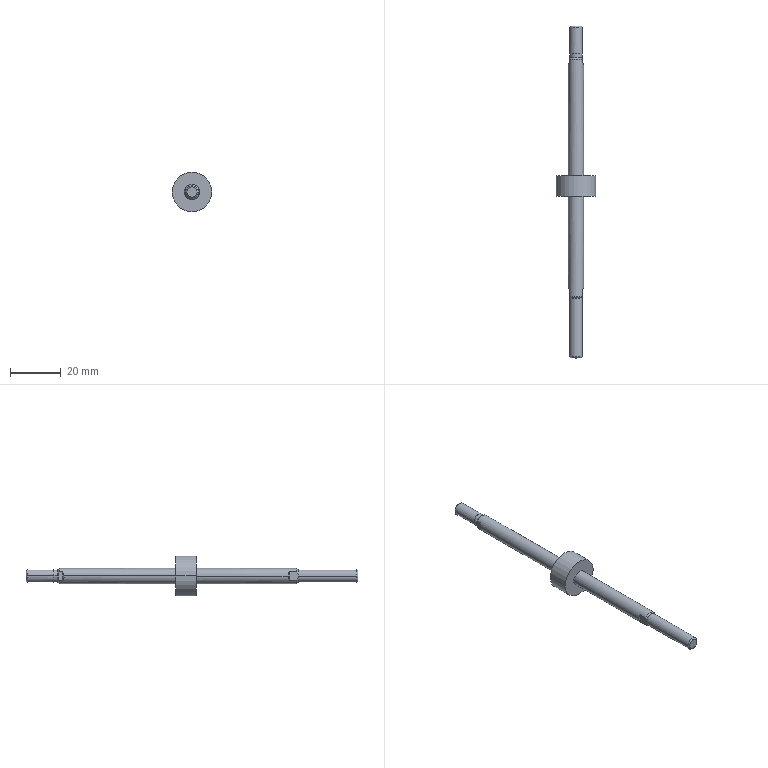Component | SolidWorks | MDJ16x20-10S_00_+-1_MDJ16x20-10S_00_+_2-1 | 1 solid | 33 faces | box 15.6 x 130.5 x 15.6 mm | volume 4691 mm3 | plane 13 | cylinder 12 | cone 8 | commonest cylinder face diameters 6 x4 5 x4 4.8 x2 15.6 x2
STEP:
#1=CARTESIAN_POINT('',(10.623,5.599,9.426));
#2=VERTEX_POINT('',#1);
#3=CARTESIAN_POINT('',(10.604,5.579,9.361));
#4=VERTEX_POINT('',#3);
#5=CARTESIAN_POINT('',(10.623,5.599,9.426));
#6=CARTESIAN_POINT('',(10.61,5.586,9.407));
#7=CARTESIAN_POINT('',(10.604,5.579,9.384));
#8=CARTESIAN_POINT('',(10.604,5.579,9.361));
#9=(BOUNDED_CURVE()B_SPLINE_CURVE(3,(#5,#6,#7,#8),.UNSPECIFIED.,.F.,.F.)B_SPLINE_CURVE_WITH_KNOTS((4,4),(5.697,6.283),.UNSPECIFIED.)CURVE()GEOMETRIC_REPRESENTATION_ITEM()RATIONAL_B_SPLINE_CURVE((1.,0.9716,0.9716,1.))REPRESENTATION_ITEM(''));
#10=EDGE_CURVE('',#2,#4,#9,.T.);
#11=ORIENTED_EDGE('',*,*,#10,.T.);
#12=CARTESIAN_POINT('',(10.604,3.855,9.361));
#13=VERTEX_POINT('',#12);
#14=CARTESIAN_POINT('',(10.604,4.754,9.361));
#15=DIRECTION('',(0.,-1.,-0.));
#16=VECTOR('',#15,39.37);
#17=LINE('',#14,#16);
#18=EDGE_CURVE('',#4,#13,#17,.T.);
#19=ORIENTED_EDGE('',*,*,#18,.T.);
#20=CARTESIAN_POINT('',(10.84,3.855,9.361));
#21=VERTEX_POINT('',#20);
#22=CARTESIAN_POINT('',(10.722,3.855,9.361));
#23=DIRECTION('',(-0.,1.,0.));
#24=DIRECTION('',(1.,0.,0.));
#25=AXIS2_PLACEMENT_3D('',#22,#23,#24);
#26=CIRCLE('',#25,0.1181);
#27=EDGE_CURVE('',#13,#21,#26,.T.);
#28=ORIENTED_EDGE('',*,*,#27,.T.);
#29=CARTESIAN_POINT('',(10.84,5.579,9.361));
#30=VERTEX_POINT('',#29);
#31=CARTESIAN_POINT('',(10.84,4.754,9.361));
#32=DIRECTION('',(0.,-1.,-0.));
#33=VECTOR('',#32,39.37);
#34=LINE('',#31,#33);
#35=EDGE_CURVE('',#30,#21,#34,.T.);
#36=ORIENTED_EDGE('',*,*,#35,.F.);
#37=CARTESIAN_POINT('',(10.82,5.599,9.426));
#38=VERTEX_POINT('',#37);
#39=CARTESIAN_POINT('',(10.84,5.579,9.361));
#40=CARTESIAN_POINT('',(10.84,5.579,9.384));
#41=CARTESIAN_POINT('',(10.833,5.586,9.407));
#42=CARTESIAN_POINT('',(10.82,5.599,9.426));
#43=(BOUNDED_CURVE()B_SPLINE_CURVE(3,(#39,#40,#41,#42),.UNSPECIFIED.,.F.,.T.)B_SPLINE_CURVE_WITH_KNOTS((4,4),(0.,0.5857),.UNSPECIFIED.)CURVE()GEOMETRIC_REPRESENTATION_ITEM()RATIONAL_B_SPLINE_CURVE((1.,0.9716,0.9716,1.))REPRESENTATION_ITEM(''));
#44=EDGE_CURVE('',#30,#38,#43,.T.);
#45=ORIENTED_EDGE('',*,*,#44,.T.);
#46=CARTESIAN_POINT('',(10.82,5.654,9.426));
#47=VERTEX_POINT('',#46);
#48=CARTESIAN_POINT('',(10.82,5.599,9.426));
#49=DIRECTION('',(-0.,1.,0.));
#50=VECTOR('',#49,39.37);
#51=LINE('',#48,#50);
#52=EDGE_CURVE('',#38,#47,#51,.T.);
#53=ORIENTED_EDGE('',*,*,#52,.T.);
#54=CARTESIAN_POINT('',(10.623,5.654,9.426));
#55=VERTEX_POINT('',#54);
#56=CARTESIAN_POINT('',(10.722,5.654,9.361));
#57=DIRECTION('',(0.,-1.,-0.));
#58=DIRECTION('',(1.,0.,0.));
#59=AXIS2_PLACEMENT_3D('',#56,#57,#58);
#60=CIRCLE('',#59,0.1181);
#61=EDGE_CURVE('',#47,#55,#60,.T.);
#62=ORIENTED_EDGE('',*,*,#61,.T.);
#63=CARTESIAN_POINT('',(10.623,5.677,9.426));
#64=DIRECTION('',(0.,-1.,-0.));
#65=VECTOR('',#64,39.37);
#66=LINE('',#63,#65);
#67=EDGE_CURVE('',#55,#2,#66,.T.);
#68=ORIENTED_EDGE('',*,*,#67,.T.);
#69=EDGE_LOOP('',(#11,#19,#28,#36,#45,#53,#62,#68));
#70=FACE_OUTER_BOUND('',#69,.T.);
#71=CARTESIAN_POINT('',(10.722,4.754,9.361));
#72=DIRECTION('',(0.,-1.,-0.));
#73=DIRECTION('',(1.,0.,0.));
#74=AXIS2_PLACEMENT_3D('',#71,#72,#73);
#75=CYLINDRICAL_SURFACE('',#74,0.1181);
#76=ADVANCED_FACE('',(#70),#75,.T.);
#77=CARTESIAN_POINT('',(10.816,5.677,9.361));
#78=VERTEX_POINT('',#77);
#79=CARTESIAN_POINT('',(10.627,5.677,9.361));
#80=VERTEX_POINT('',#79);
#81=CARTESIAN_POINT('',(10.722,5.677,9.361));
#82=DIRECTION('',(0.,-1.,-0.));
#83=DIRECTION('',(-1.,0.,0.));
#84=AXIS2_PLACEMENT_3D('',#81,#82,#83);
#85=CIRCLE('',#84,0.09449);
#86=EDGE_CURVE('',#78,#80,#85,.T.);
#87=ORIENTED_EDGE('',*,*,#86,.T.);
#88=CARTESIAN_POINT('',(10.623,5.673,9.361));
#89=VERTEX_POINT('',#88);
#90=CARTESIAN_POINT('',(10.604,5.654,9.361));
#91=DIRECTION('',(-0.7071,-0.7071,-0.));
#92=VECTOR('',#91,39.37);
#93=LINE('',#90,#92);
#94=EDGE_CURVE('',#80,#89,#93,.T.);
#95=ORIENTED_EDGE('',*,*,#94,.T.);
#96=CARTESIAN_POINT('',(10.623,5.673,9.361));
#97=CARTESIAN_POINT('',(10.623,5.673,9.372));
#98=CARTESIAN_POINT('',(10.623,5.671,9.384));
#99=CARTESIAN_POINT('',(10.623,5.664,9.406));
#100=CARTESIAN_POINT('',(10.623,5.659,9.416));
#101=CARTESIAN_POINT('',(10.623,5.654,9.426));
#102=B_SPLINE_CURVE_WITH_KNOTS('',3,(#96,#97,#98,#99,#100,#101),.UNSPECIFIED.,.F.,.F.,(4,2,4),(0.,0.0008701,0.00174),.UNSPECIFIED.);
#103=EDGE_CURVE('',#89,#55,#102,.T.);
#104=ORIENTED_EDGE('',*,*,#103,.T.);
#105=ORIENTED_EDGE('',*,*,#61,.F.);
#106=CARTESIAN_POINT('',(10.82,5.673,9.361));
#107=VERTEX_POINT('',#106);
#108=CARTESIAN_POINT('',(10.82,5.654,9.426));
#109=CARTESIAN_POINT('',(10.82,5.659,9.416));
#110=CARTESIAN_POINT('',(10.82,5.664,9.406));
#111=CARTESIAN_POINT('',(10.82,5.671,9.384));
#112=CARTESIAN_POINT('',(10.82,5.673,9.372));
#113=CARTESIAN_POINT('',(10.82,5.673,9.361));
#114=B_SPLINE_CURVE_WITH_KNOTS('',3,(#108,#109,#110,#111,#112,#113),.UNSPECIFIED.,.F.,.F.,(4,2,4),(0.,0.0008701,0.00174),.UNSPECIFIED.);
#115=EDGE_CURVE('',#47,#107,#114,.T.);
#116=ORIENTED_EDGE('',*,*,#115,.T.);
#117=CARTESIAN_POINT('',(10.84,5.654,9.361));
#118=DIRECTION('',(0.7071,-0.7071,-0.));
#119=VECTOR('',#118,39.37);
#120=LINE('',#117,#119);
#121=EDGE_CURVE('',#78,#107,#120,.T.);
#122=ORIENTED_EDGE('',*,*,#121,.F.);
#123=EDGE_LOOP('',(#87,#95,#104,#105,#116,#122));
#124=FACE_OUTER_BOUND('',#123,.T.);
#125=CARTESIAN_POINT('',(10.722,5.654,9.361));
#126=DIRECTION('',(0.,-1.,-0.));
#127=DIRECTION('',(1.,0.,0.));
#128=AXIS2_PLACEMENT_3D('',#125,#126,#127);
#129=CONICAL_SURFACE('',#128,0.1181,0.7854);
#130=ADVANCED_FACE('',(#124),#129,.T.);
#131=CARTESIAN_POINT('',(10.816,5.736,9.361));
#132=VERTEX_POINT('',#131);
#133=CARTESIAN_POINT('',(10.627,5.736,9.361));
#134=VERTEX_POINT('',#133);
#135=CARTESIAN_POINT('',(10.722,5.736,9.361));
#136=DIRECTION('',(0.,-1.,-0.));
#137=DIRECTION('',(1.,0.,0.));
#138=AXIS2_PLACEMENT_3D('',#135,#136,#137);
#139=CIRCLE('',#138,0.09449);
#140=EDGE_CURVE('',#132,#134,#139,.T.);
#141=ORIENTED_EDGE('',*,*,#140,.T.);
#142=CARTESIAN_POINT('',(10.627,5.707,9.361));
#143=DIRECTION('',(0.,-1.,-0.));
#144=VECTOR('',#143,39.37);
#145=LINE('',#142,#144);
#146=EDGE_CURVE('',#134,#80,#145,.T.);
#147=ORIENTED_EDGE('',*,*,#146,.T.);
#148=ORIENTED_EDGE('',*,*,#86,.F.);
#149=CARTESIAN_POINT('',(10.816,5.707,9.361));
#150=DIRECTION('',(0.,-1.,-0.));
#151=VECTOR('',#150,39.37);
#152=LINE('',#149,#151);
#153=EDGE_CURVE('',#132,#78,#152,.T.);
#154=ORIENTED_EDGE('',*,*,#153,.F.);
#155=EDGE_LOOP('',(#141,#147,#148,#154));
#156=FACE_OUTER_BOUND('',#155,.T.);
#157=CARTESIAN_POINT('',(10.722,5.707,9.361));
#158=DIRECTION('',(0.,-1.,-0.));
#159=DIRECTION('',(1.,0.,0.));
#160=AXIS2_PLACEMENT_3D('',#157,#158,#159);
#161=CYLINDRICAL_SURFACE('',#160,0.09449);
#162=ADVANCED_FACE('',(#156),#161,.T.);
#163=CARTESIAN_POINT('',(10.415,3.855,9.361));
#164=VERTEX_POINT('',#163);
#165=CARTESIAN_POINT('',(11.029,3.855,9.361));
#166=VERTEX_POINT('',#165);
#167=CARTESIAN_POINT('',(10.722,3.855,9.361));
#168=DIRECTION('',(-0.,1.,0.));
#169=DIRECTION('',(1.,0.,0.));
#170=AXIS2_PLACEMENT_3D('',#167,#168,#169);
#171=CIRCLE('',#170,0.3071);
#172=EDGE_CURVE('',#164,#166,#171,.T.);
#173=ORIENTED_EDGE('',*,*,#172,.F.);
#174=CARTESIAN_POINT('',(10.415,3.532,9.361));
#175=VERTEX_POINT('',#174);
#176=CARTESIAN_POINT('',(10.415,3.693,9.361));
#177=DIRECTION('',(0.,-1.,-0.));
#178=VECTOR('',#177,39.37);
#179=LINE('',#176,#178);
#180=EDGE_CURVE('',#164,#175,#179,.T.);
#181=ORIENTED_EDGE('',*,*,#180,.T.);
#182=CARTESIAN_POINT('',(11.029,3.532,9.361));
#183=VERTEX_POINT('',#182);
#184=CARTESIAN_POINT('',(10.722,3.532,9.361));
#185=DIRECTION('',(-0.,1.,0.));
#186=DIRECTION('',(1.,0.,0.));
#187=AXIS2_PLACEMENT_3D('',#184,#185,#186);
#188=CIRCLE('',#187,0.3071);
#189=EDGE_CURVE('',#175,#183,#188,.T.);
#190=ORIENTED_EDGE('',*,*,#189,.T.);
#191=CARTESIAN_POINT('',(11.029,3.693,9.361));
#192=DIRECTION('',(0.,-1.,-0.));
#193=VECTOR('',#192,39.37);
#194=LINE('',#191,#193);
#195=EDGE_CURVE('',#166,#183,#194,.T.);
#196=ORIENTED_EDGE('',*,*,#195,.F.);
#197=EDGE_LOOP('',(#173,#181,#190,#196));
#198=FACE_OUTER_BOUND('',#197,.T.);
#199=CARTESIAN_POINT('',(10.722,3.693,9.361));
#200=DIRECTION('',(0.,-1.,-0.));
#201=DIRECTION('',(1.,0.,0.));
#202=AXIS2_PLACEMENT_3D('',#199,#200,#201);
#203=CYLINDRICAL_SURFACE('',#202,0.3071);
#204=ADVANCED_FACE('',(#198),#203,.T.);
#205=CARTESIAN_POINT('',(10.722,6.15,9.459));
#206=VERTEX_POINT('',#205);
#207=CARTESIAN_POINT('',(10.623,6.15,9.361));
#208=VERTEX_POINT('',#207);
#209=CARTESIAN_POINT('',(10.722,6.15,9.361));
#210=DIRECTION('',(0.,-1.,-0.));
#211=DIRECTION('',(1.,0.,0.));
#212=AXIS2_PLACEMENT_3D('',#209,#210,#211);
#213=CIRCLE('',#212,0.09843);
#214=EDGE_CURVE('',#206,#208,#213,.T.);
#215=ORIENTED_EDGE('',*,*,#214,.T.);
#216=CARTESIAN_POINT('',(10.623,5.736,9.361));
#217=VERTEX_POINT('',#216);
#218=CARTESIAN_POINT('',(10.623,5.943,9.361));
#219=DIRECTION('',(0.,-1.,-0.));
#220=VECTOR('',#219,39.37);
#221=LINE('',#218,#220);
#222=EDGE_CURVE('',#208,#217,#221,.T.);
#223=ORIENTED_EDGE('',*,*,#222,.T.);
#224=CARTESIAN_POINT('',(10.82,5.736,9.361));
#225=VERTEX_POINT('',#224);
#226=CARTESIAN_POINT('',(10.722,5.736,9.361));
#227=DIRECTION('',(0.,-1.,-0.));
#228=DIRECTION('',(1.,0.,0.));
#229=AXIS2_PLACEMENT_3D('',#226,#227,#228);
#230=CIRCLE('',#229,0.09843);
#231=EDGE_CURVE('',#225,#217,#230,.T.);
#232=ORIENTED_EDGE('',*,*,#231,.F.);
#233=CARTESIAN_POINT('',(10.82,6.15,9.361));
#234=VERTEX_POINT('',#233);
#235=CARTESIAN_POINT('',(10.82,5.943,9.361));
#236=DIRECTION('',(0.,-1.,-0.));
#237=VECTOR('',#236,39.37);
#238=LINE('',#235,#237);
#239=EDGE_CURVE('',#234,#225,#238,.T.);
#240=ORIENTED_EDGE('',*,*,#239,.F.);
#241=CARTESIAN_POINT('',(10.722,6.15,9.361));
#242=DIRECTION('',(0.,-1.,-0.));
#243=DIRECTION('',(1.,0.,0.));
#244=AXIS2_PLACEMENT_3D('',#241,#242,#243);
#245=CIRCLE('',#244,0.09843);
#246=EDGE_CURVE('',#234,#206,#245,.T.);
#247=ORIENTED_EDGE('',*,*,#246,.T.);
#248=EDGE_LOOP('',(#215,#223,#232,#240,#247));
#249=FACE_OUTER_BOUND('',#248,.T.);
#250=CARTESIAN_POINT('',(10.722,5.943,9.361));
#251=DIRECTION('',(0.,-1.,-0.));
#252=DIRECTION('',(1.,0.,0.));
#253=AXIS2_PLACEMENT_3D('',#250,#251,#252);
#254=CYLINDRICAL_SURFACE('',#253,0.09843);
#255=ADVANCED_FACE('',(#249),#254,.T.);
#256=CARTESIAN_POINT('',(10.604,3.532,9.361));
#257=VERTEX_POINT('',#256);
#258=CARTESIAN_POINT('',(10.84,3.532,9.361));
#259=VERTEX_POINT('',#258);
#260=CARTESIAN_POINT('',(10.722,3.532,9.361));
#261=DIRECTION('',(-0.,1.,0.));
#262=DIRECTION('',(1.,0.,0.));
#263=AXIS2_PLACEMENT_3D('',#260,#261,#262);
#264=CIRCLE('',#263,0.1181);
#265=EDGE_CURVE('',#257,#259,#264,.T.);
#266=ORIENTED_EDGE('',*,*,#265,.F.);
#267=CARTESIAN_POINT('',(10.604,2.114,9.361));
#268=VERTEX_POINT('',#267);
#269=CARTESIAN_POINT('',(10.604,2.754,9.361));
#270=DIRECTION('',(0.,-1.,-0.));
#271=VECTOR('',#270,39.37);
#272=LINE('',#269,#271);
#273=EDGE_CURVE('',#257,#268,#272,.T.);
#274=ORIENTED_EDGE('',*,*,#273,.T.);
#275=CARTESIAN_POINT('',(10.623,2.095,9.426));
#276=VERTEX_POINT('',#275);
#277=CARTESIAN_POINT('',(10.604,2.114,9.361));
#278=CARTESIAN_POINT('',(10.604,2.114,9.384));
#279=CARTESIAN_POINT('',(10.61,2.108,9.407));
#280=CARTESIAN_POINT('',(10.623,2.095,9.426));
#281=(BOUNDED_CURVE()B_SPLINE_CURVE(3,(#277,#278,#279,#280),.UNSPECIFIED.,.F.,.T.)B_SPLINE_CURVE_WITH_KNOTS((4,4),(3.142,3.727),.UNSPECIFIED.)CURVE()GEOMETRIC_REPRESENTATION_ITEM()RATIONAL_B_SPLINE_CURVE((1.,0.9716,0.9716,1.))REPRESENTATION_ITEM(''));
#282=EDGE_CURVE('',#268,#276,#281,.T.);
#283=ORIENTED_EDGE('',*,*,#282,.T.);
#284=CARTESIAN_POINT('',(10.623,1.977,9.426));
#285=VERTEX_POINT('',#284);
#286=CARTESIAN_POINT('',(10.623,2.754,9.426));
#287=DIRECTION('',(0.,-1.,-0.));
#288=VECTOR('',#287,39.37);
#289=LINE('',#286,#288);
#290=EDGE_CURVE('',#276,#285,#289,.T.);
#291=ORIENTED_EDGE('',*,*,#290,.T.);
#292=CARTESIAN_POINT('',(10.82,1.977,9.426));
#293=VERTEX_POINT('',#292);
#294=CARTESIAN_POINT('',(10.722,1.977,9.361));
#295=DIRECTION('',(-0.,1.,0.));
#296=DIRECTION('',(1.,0.,-0.));
#297=AXIS2_PLACEMENT_3D('',#294,#295,#296);
#298=CIRCLE('',#297,0.1181);
#299=EDGE_CURVE('',#285,#293,#298,.T.);
#300=ORIENTED_EDGE('',*,*,#299,.T.);
#301=CARTESIAN_POINT('',(10.82,2.095,9.426));
#302=VERTEX_POINT('',#301);
#303=CARTESIAN_POINT('',(10.82,2.754,9.426));
#304=DIRECTION('',(-0.,1.,0.));
#305=VECTOR('',#304,39.37);
#306=LINE('',#303,#305);
#307=EDGE_CURVE('',#293,#302,#306,.T.);
#308=ORIENTED_EDGE('',*,*,#307,.T.);
#309=CARTESIAN_POINT('',(10.84,2.114,9.361));
#310=VERTEX_POINT('',#309);
#311=CARTESIAN_POINT('',(10.82,2.095,9.426));
#312=CARTESIAN_POINT('',(10.833,2.108,9.407));
#313=CARTESIAN_POINT('',(10.84,2.114,9.384));
#314=CARTESIAN_POINT('',(10.84,2.114,9.361));
#315=(BOUNDED_CURVE()B_SPLINE_CURVE(3,(#311,#312,#313,#314),.UNSPECIFIED.,.F.,.F.)B_SPLINE_CURVE_WITH_KNOTS((4,4),(2.556,3.142),.UNSPECIFIED.)CURVE()GEOMETRIC_REPRESENTATION_ITEM()RATIONAL_B_SPLINE_CURVE((1.,0.9716,0.9716,1.))REPRESENTATION_ITEM(''));
#316=EDGE_CURVE('',#302,#310,#315,.T.);
#317=ORIENTED_EDGE('',*,*,#316,.T.);
#318=CARTESIAN_POINT('',(10.84,2.754,9.361));
#319=DIRECTION('',(0.,-1.,-0.));
#320=VECTOR('',#319,39.37);
#321=LINE('',#318,#320);
#322=EDGE_CURVE('',#259,#310,#321,.T.);
#323=ORIENTED_EDGE('',*,*,#322,.F.);
#324=EDGE_LOOP('',(#266,#274,#283,#291,#300,#308,#317,#323));
#325=FACE_OUTER_BOUND('',#324,.T.);
#326=CARTESIAN_POINT('',(10.722,2.754,9.361));
#327=DIRECTION('',(0.,-1.,-0.));
#328=DIRECTION('',(1.,0.,0.));
#329=AXIS2_PLACEMENT_3D('',#326,#327,#328);
#330=CYLINDRICAL_SURFACE('',#329,0.1181);
#331=ADVANCED_FACE('',(#325),#330,.T.);
#332=CARTESIAN_POINT('',(10.722,6.169,9.44));
#333=VERTEX_POINT('',#332);
#334=CARTESIAN_POINT('',(10.722,6.169,9.282));
#335=VERTEX_POINT('',#334);
#336=CARTESIAN_POINT('',(10.722,6.169,9.361));
#337=DIRECTION('',(0.,-1.,0.));
#338=DIRECTION('',(0.,0.,1.));
#339=AXIS2_PLACEMENT_3D('',#336,#337,#338);
#340=CIRCLE('',#339,0.07911);
#341=EDGE_CURVE('',#333,#335,#340,.T.);
#342=ORIENTED_EDGE('',*,*,#341,.T.);
#343=CARTESIAN_POINT('',(10.722,6.15,9.262));
#344=VERTEX_POINT('',#343);
#345=CARTESIAN_POINT('',(10.722,6.15,9.262));
#346=DIRECTION('',(-0.,-0.7071,-0.7071));
#347=VECTOR('',#346,39.37);
#348=LINE('',#345,#347);
#349=EDGE_CURVE('',#335,#344,#348,.T.);
#350=ORIENTED_EDGE('',*,*,#349,.T.);
#351=CARTESIAN_POINT('',(10.722,6.15,9.361));
#352=DIRECTION('',(0.,-1.,-0.));
#353=DIRECTION('',(1.,0.,0.));
#354=AXIS2_PLACEMENT_3D('',#351,#352,#353);
#355=CIRCLE('',#354,0.09843);
#356=EDGE_CURVE('',#208,#344,#355,.T.);
#357=ORIENTED_EDGE('',*,*,#356,.F.);
#358=ORIENTED_EDGE('',*,*,#214,.F.);
#359=CARTESIAN_POINT('',(10.722,6.15,9.459));
#360=DIRECTION('',(0.,-0.7071,0.7071));
#361=VECTOR('',#360,39.37);
#362=LINE('',#359,#361);
#363=EDGE_CURVE('',#333,#206,#362,.T.);
#364=ORIENTED_EDGE('',*,*,#363,.F.);
#365=EDGE_LOOP('',(#342,#350,#357,#358,#364));
#366=FACE_OUTER_BOUND('',#365,.T.);
#367=CARTESIAN_POINT('',(10.722,6.15,9.361));
#368=DIRECTION('',(0.,-1.,0.));
#369=DIRECTION('',(0.,0.,1.));
#370=AXIS2_PLACEMENT_3D('',#367,#368,#369);
#371=CONICAL_SURFACE('',#370,0.09843,0.7854);
#372=ADVANCED_FACE('',(#366),#371,.T.);
#373=CARTESIAN_POINT('',(10.623,1.957,9.361));
#374=VERTEX_POINT('',#373);
#375=CARTESIAN_POINT('',(10.82,1.957,9.361));
#376=VERTEX_POINT('',#375);
#377=CARTESIAN_POINT('',(10.722,1.957,9.361));
#378=DIRECTION('',(-0.,1.,0.));
#379=DIRECTION('',(-1.,0.,0.));
#380=AXIS2_PLACEMENT_3D('',#377,#378,#379);
#381=CIRCLE('',#380,0.09843);
#382=EDGE_CURVE('',#374,#376,#381,.T.);
#383=ORIENTED_EDGE('',*,*,#382,.F.);
#384=CARTESIAN_POINT('',(10.623,1.051,9.361));
#385=VERTEX_POINT('',#384);
#386=CARTESIAN_POINT('',(10.623,1.504,9.361));
#387=DIRECTION('',(0.,-1.,-0.));
#388=VECTOR('',#387,39.37);
#389=LINE('',#386,#388);
#390=EDGE_CURVE('',#374,#385,#389,.T.);
#391=ORIENTED_EDGE('',*,*,#390,.T.);
#392=CARTESIAN_POINT('',(10.82,1.051,9.361));
#393=VERTEX_POINT('',#392);
#394=CARTESIAN_POINT('',(10.722,1.051,9.361));
#395=DIRECTION('',(-0.,1.,0.));
#396=DIRECTION('',(1.,0.,0.));
#397=AXIS2_PLACEMENT_3D('',#394,#395,#396);
#398=CIRCLE('',#397,0.09843);
#399=EDGE_CURVE('',#385,#393,#398,.T.);
#400=ORIENTED_EDGE('',*,*,#399,.T.);
#401=CARTESIAN_POINT('',(10.82,1.504,9.361));
#402=DIRECTION('',(0.,-1.,-0.));
#403=VECTOR('',#402,39.37);
#404=LINE('',#401,#403);
#405=EDGE_CURVE('',#376,#393,#404,.T.);
#406=ORIENTED_EDGE('',*,*,#405,.F.);
#407=EDGE_LOOP('',(#383,#391,#400,#406));
#408=FACE_OUTER_BOUND('',#407,.T.);
#409=CARTESIAN_POINT('',(10.722,1.504,9.361));
#410=DIRECTION('',(0.,-1.,-0.));
#411=DIRECTION('',(1.,0.,0.));
#412=AXIS2_PLACEMENT_3D('',#409,#410,#411);
#413=CYLINDRICAL_SURFACE('',#412,0.09843);
#414=ADVANCED_FACE('',(#408),#413,.T.);
#415=CARTESIAN_POINT('',(10.643,1.032,9.361));
#416=VERTEX_POINT('',#415);
#417=CARTESIAN_POINT('',(10.801,1.032,9.361));
#418=VERTEX_POINT('',#417);
#419=CARTESIAN_POINT('',(10.722,1.032,9.361));
#420=DIRECTION('',(-0.,1.,0.));
#421=DIRECTION('',(-1.,0.,0.));
#422=AXIS2_PLACEMENT_3D('',#419,#420,#421);
#423=CIRCLE('',#422,0.07911);
#424=EDGE_CURVE('',#416,#418,#423,.T.);
#425=ORIENTED_EDGE('',*,*,#424,.T.);
#426=CARTESIAN_POINT('',(10.82,1.051,9.361));
#427=DIRECTION('',(0.7071,0.7071,0.));
#428=VECTOR('',#427,39.37);
#429=LINE('',#426,#428);
#430=EDGE_CURVE('',#418,#393,#429,.T.);
#431=ORIENTED_EDGE('',*,*,#430,.T.);
#432=ORIENTED_EDGE('',*,*,#399,.F.);
#433=CARTESIAN_POINT('',(10.623,1.051,9.361));
#434=DIRECTION('',(-0.7071,0.7071,0.));
#435=VECTOR('',#434,39.37);
#436=LINE('',#433,#435);
#437=EDGE_CURVE('',#416,#385,#436,.T.);
#438=ORIENTED_EDGE('',*,*,#437,.F.);
#439=EDGE_LOOP('',(#425,#431,#432,#438));
#440=FACE_OUTER_BOUND('',#439,.T.);
#441=CARTESIAN_POINT('',(10.722,1.051,9.361));
#442=DIRECTION('',(-0.,1.,0.));
#443=DIRECTION('',(-1.,0.,0.));
#444=AXIS2_PLACEMENT_3D('',#441,#442,#443);
#445=CONICAL_SURFACE('',#444,0.09843,0.7854);
#446=ADVANCED_FACE('',(#440),#445,.T.);
#447=ORIENTED_EDGE('',*,*,#18,.F.);
#448=CARTESIAN_POINT('',(10.623,5.599,9.296));
#449=VERTEX_POINT('',#448);
#450=CARTESIAN_POINT('',(10.604,5.579,9.361));
#451=CARTESIAN_POINT('',(10.604,5.579,9.337));
#452=CARTESIAN_POINT('',(10.61,5.586,9.315));
#453=CARTESIAN_POINT('',(10.623,5.599,9.296));
#454=(BOUNDED_CURVE()B_SPLINE_CURVE(3,(#450,#451,#452,#453),.UNSPECIFIED.,.F.,.F.)B_SPLINE_CURVE_WITH_KNOTS((4,4),(0.,0.5857),.UNSPECIFIED.)CURVE()GEOMETRIC_REPRESENTATION_ITEM()RATIONAL_B_SPLINE_CURVE((1.,0.9716,0.9716,1.))REPRESENTATION_ITEM(''));
#455=EDGE_CURVE('',#4,#449,#454,.T.);
#456=ORIENTED_EDGE('',*,*,#455,.T.);
#457=CARTESIAN_POINT('',(10.623,5.654,9.296));
#458=VERTEX_POINT('',#457);
#459=CARTESIAN_POINT('',(10.623,4.754,9.296));
#460=DIRECTION('',(-0.,1.,0.));
#461=VECTOR('',#460,39.37);
#462=LINE('',#459,#461);
#463=EDGE_CURVE('',#449,#458,#462,.T.);
#464=ORIENTED_EDGE('',*,*,#463,.T.);
#465=CARTESIAN_POINT('',(10.82,5.654,9.296));
#466=VERTEX_POINT('',#465);
#467=CARTESIAN_POINT('',(10.722,5.654,9.361));
#468=DIRECTION('',(0.,-1.,-0.));
#469=DIRECTION('',(1.,0.,0.));
#470=AXIS2_PLACEMENT_3D('',#467,#468,#469);
#471=CIRCLE('',#470,0.1181);
#472=EDGE_CURVE('',#458,#466,#471,.T.);
#473=ORIENTED_EDGE('',*,*,#472,.T.);
#474=CARTESIAN_POINT('',(10.82,5.599,9.296));
#475=VERTEX_POINT('',#474);
#476=CARTESIAN_POINT('',(10.82,4.754,9.296));
#477=DIRECTION('',(0.,-1.,-0.));
#478=VECTOR('',#477,39.37);
#479=LINE('',#476,#478);
#480=EDGE_CURVE('',#466,#475,#479,.T.);
#481=ORIENTED_EDGE('',*,*,#480,.T.);
#482=CARTESIAN_POINT('',(10.82,5.599,9.296));
#483=CARTESIAN_POINT('',(10.833,5.586,9.315));
#484=CARTESIAN_POINT('',(10.84,5.579,9.337));
#485=CARTESIAN_POINT('',(10.84,5.579,9.361));
#486=(BOUNDED_CURVE()B_SPLINE_CURVE(3,(#482,#483,#484,#485),.UNSPECIFIED.,.F.,.T.)B_SPLINE_CURVE_WITH_KNOTS((4,4),(5.697,6.283),.UNSPECIFIED.)CURVE()GEOMETRIC_REPRESENTATION_ITEM()RATIONAL_B_SPLINE_CURVE((1.,0.9716,0.9716,1.))REPRESENTATION_ITEM(''));
#487=EDGE_CURVE('',#475,#30,#486,.T.);
#488=ORIENTED_EDGE('',*,*,#487,.T.);
#489=ORIENTED_EDGE('',*,*,#35,.T.);
#490=CARTESIAN_POINT('',(10.722,3.855,9.361));
#491=DIRECTION('',(-0.,1.,0.));
#492=DIRECTION('',(1.,0.,0.));
#493=AXIS2_PLACEMENT_3D('',#490,#491,#492);
#494=CIRCLE('',#493,0.1181);
#495=EDGE_CURVE('',#21,#13,#494,.T.);
#496=ORIENTED_EDGE('',*,*,#495,.T.);
#497=EDGE_LOOP('',(#447,#456,#464,#473,#481,#488,#489,#496));
#498=FACE_OUTER_BOUND('',#497,.T.);
#499=CARTESIAN_POINT('',(10.722,4.754,9.361));
#500=DIRECTION('',(0.,-1.,-0.));
#501=DIRECTION('',(1.,0.,0.));
#502=AXIS2_PLACEMENT_3D('',#499,#500,#501);
#503=CYLINDRICAL_SURFACE('',#502,0.1181);
#504=ADVANCED_FACE('',(#498),#503,.T.);
#505=CARTESIAN_POINT('',(10.623,5.599,9.125));
#506=DIRECTION('',(0.,-0.,1.));
#507=VECTOR('',#506,39.37);
#508=LINE('',#505,#507);
#509=EDGE_CURVE('',#449,#2,#508,.T.);
#510=ORIENTED_EDGE('',*,*,#509,.F.);
#511=ORIENTED_EDGE('',*,*,#455,.F.);
#512=ORIENTED_EDGE('',*,*,#10,.F.);
#513=EDGE_LOOP('',(#510,#511,#512));
#514=FACE_OUTER_BOUND('',#513,.T.);
#515=CARTESIAN_POINT('',(10.623,5.599,9.125));
#516=DIRECTION('',(0.7071,-0.7071,-0.));
#517=DIRECTION('',(0.7071,0.7071,0.));
#518=AXIS2_PLACEMENT_3D('',#515,#516,#517);
#519=PLANE('',#518);
#520=ADVANCED_FACE('',(#514),#519,.F.);
#521=ORIENTED_EDGE('',*,*,#94,.F.);
#522=CARTESIAN_POINT('',(10.722,5.677,9.361));
#523=DIRECTION('',(0.,-1.,-0.));
#524=DIRECTION('',(-1.,0.,0.));
#525=AXIS2_PLACEMENT_3D('',#522,#523,#524);
#526=CIRCLE('',#525,0.09449);
#527=EDGE_CURVE('',#80,#78,#526,.T.);
#528=ORIENTED_EDGE('',*,*,#527,.T.);
#529=ORIENTED_EDGE('',*,*,#121,.T.);
#530=CARTESIAN_POINT('',(10.82,5.673,9.361));
#531=CARTESIAN_POINT('',(10.82,5.673,9.349));
#532=CARTESIAN_POINT('',(10.82,5.671,9.338));
#533=CARTESIAN_POINT('',(10.82,5.664,9.316));
#534=CARTESIAN_POINT('',(10.82,5.659,9.306));
#535=CARTESIAN_POINT('',(10.82,5.654,9.296));
#536=B_SPLINE_CURVE_WITH_KNOTS('',3,(#530,#531,#532,#533,#534,#535),.UNSPECIFIED.,.F.,.F.,(4,2,4),(0.00174,0.00261,0.003479),.UNSPECIFIED.);
#537=EDGE_CURVE('',#107,#466,#536,.T.);
#538=ORIENTED_EDGE('',*,*,#537,.T.);
#539=ORIENTED_EDGE('',*,*,#472,.F.);
#540=CARTESIAN_POINT('',(10.623,5.654,9.296));
#541=CARTESIAN_POINT('',(10.623,5.659,9.306));
#542=CARTESIAN_POINT('',(10.623,5.664,9.316));
#543=CARTESIAN_POINT('',(10.623,5.671,9.338));
#544=CARTESIAN_POINT('',(10.623,5.673,9.349));
#545=CARTESIAN_POINT('',(10.623,5.673,9.361));
#546=B_SPLINE_CURVE_WITH_KNOTS('',3,(#540,#541,#542,#543,#544,#545),.UNSPECIFIED.,.F.,.F.,(4,2,4),(-0.001741,-0.0008706,0.),.UNSPECIFIED.);
#547=EDGE_CURVE('',#458,#89,#546,.T.);
#548=ORIENTED_EDGE('',*,*,#547,.T.);
#549=EDGE_LOOP('',(#521,#528,#529,#538,#539,#548));
#550=FACE_OUTER_BOUND('',#549,.T.);
#551=CARTESIAN_POINT('',(10.722,5.654,9.361));
#552=DIRECTION('',(0.,-1.,-0.));
#553=DIRECTION('',(1.,0.,0.));
#554=AXIS2_PLACEMENT_3D('',#551,#552,#553);
#555=CONICAL_SURFACE('',#554,0.1181,0.7854);
#556=ADVANCED_FACE('',(#550),#555,.T.);
#557=CARTESIAN_POINT('',(10.82,5.599,9.125));
#558=DIRECTION('',(-0.,0.,-1.));
#559=VECTOR('',#558,39.37);
#560=LINE('',#557,#559);
#561=EDGE_CURVE('',#38,#475,#560,.T.);
#562=ORIENTED_EDGE('',*,*,#561,.F.);
#563=ORIENTED_EDGE('',*,*,#44,.F.);
#564=ORIENTED_EDGE('',*,*,#487,.F.);
#565=EDGE_LOOP('',(#562,#563,#564));
#566=FACE_OUTER_BOUND('',#565,.T.);
#567=CARTESIAN_POINT('',(10.958,5.461,9.125));
#568=DIRECTION('',(-0.7071,-0.7071,-0.));
#569=DIRECTION('',(0.7071,-0.7071,-0.));
#570=AXIS2_PLACEMENT_3D('',#567,#568,#569);
#571=PLANE('',#570);
#572=ADVANCED_FACE('',(#566),#571,.F.);
#573=CARTESIAN_POINT('',(10.722,3.855,9.361));
#574=DIRECTION('',(-0.,1.,0.));
#575=DIRECTION('',(1.,0.,0.));
#576=AXIS2_PLACEMENT_3D('',#573,#574,#575);
#577=CIRCLE('',#576,0.3071);
#578=EDGE_CURVE('',#166,#164,#577,.T.);
#579=ORIENTED_EDGE('',*,*,#578,.T.);
#580=ORIENTED_EDGE('',*,*,#172,.T.);
#581=EDGE_LOOP('',(#579,#580));
#582=FACE_OUTER_BOUND('',#581,.T.);
#583=ORIENTED_EDGE('',*,*,#495,.F.);
#584=ORIENTED_EDGE('',*,*,#27,.F.);
#585=EDGE_LOOP('',(#583,#584));
#586=FACE_BOUND('',#585,.T.);
#587=CARTESIAN_POINT('',(10.509,3.855,9.361));
#588=DIRECTION('',(-0.,1.,0.));
#589=DIRECTION('',(-1.,-0.,0.));
#590=AXIS2_PLACEMENT_3D('',#587,#588,#589);
#591=PLANE('',#590);
#592=ADVANCED_FACE('',(#582,#586),#591,.T.);
#593=ORIENTED_EDGE('',*,*,#547,.F.);
#594=ORIENTED_EDGE('',*,*,#463,.F.);
#595=ORIENTED_EDGE('',*,*,#509,.T.);
#596=ORIENTED_EDGE('',*,*,#67,.F.);
#597=ORIENTED_EDGE('',*,*,#103,.F.);
#598=EDGE_LOOP('',(#593,#594,#595,#596,#597));
#599=FACE_OUTER_BOUND('',#598,.T.);
#600=CARTESIAN_POINT('',(10.623,5.677,9.125));
#601=DIRECTION('',(1.,0.,-0.));
#602=DIRECTION('',(-0.,1.,0.));
#603=AXIS2_PLACEMENT_3D('',#600,#601,#602);
#604=PLANE('',#603);
#605=ADVANCED_FACE('',(#599),#604,.F.);
#606=ORIENTED_EDGE('',*,*,#146,.F.);
#607=CARTESIAN_POINT('',(10.722,5.736,9.361));
#608=DIRECTION('',(0.,-1.,-0.));
#609=DIRECTION('',(1.,0.,0.));
#610=AXIS2_PLACEMENT_3D('',#607,#608,#609);
#611=CIRCLE('',#610,0.09449);
#612=EDGE_CURVE('',#134,#132,#611,.T.);
#613=ORIENTED_EDGE('',*,*,#612,.T.);
#614=ORIENTED_EDGE('',*,*,#153,.T.);
#615=ORIENTED_EDGE('',*,*,#527,.F.);
#616=EDGE_LOOP('',(#606,#613,#614,#615));
#617=FACE_OUTER_BOUND('',#616,.T.);
#618=CARTESIAN_POINT('',(10.722,5.707,9.361));
#619=DIRECTION('',(0.,-1.,-0.));
#620=DIRECTION('',(1.,0.,0.));
#621=AXIS2_PLACEMENT_3D('',#618,#619,#620);
#622=CYLINDRICAL_SURFACE('',#621,0.09449);
#623=ADVANCED_FACE('',(#617),#622,.T.);
#624=ORIENTED_EDGE('',*,*,#561,.T.);
#625=ORIENTED_EDGE('',*,*,#480,.F.);
#626=ORIENTED_EDGE('',*,*,#537,.F.);
#627=ORIENTED_EDGE('',*,*,#115,.F.);
#628=ORIENTED_EDGE('',*,*,#52,.F.);
#629=EDGE_LOOP('',(#624,#625,#626,#627,#628));
#630=FACE_OUTER_BOUND('',#629,.T.);
#631=CARTESIAN_POINT('',(10.82,5.599,9.125));
#632=DIRECTION('',(-1.,-0.,0.));
#633=DIRECTION('',(0.,-1.,-0.));
#634=AXIS2_PLACEMENT_3D('',#631,#632,#633);
#635=PLANE('',#634);
#636=ADVANCED_FACE('',(#630),#635,.F.);
#637=ORIENTED_EDGE('',*,*,#180,.F.);
#638=ORIENTED_EDGE('',*,*,#578,.F.);
#639=ORIENTED_EDGE('',*,*,#195,.T.);
#640=CARTESIAN_POINT('',(10.722,3.532,9.361));
#641=DIRECTION('',(-0.,1.,0.));
#642=DIRECTION('',(1.,0.,0.));
#643=AXIS2_PLACEMENT_3D('',#640,#641,#642);
#644=CIRCLE('',#643,0.3071);
#645=EDGE_CURVE('',#183,#175,#644,.T.);
#646=ORIENTED_EDGE('',*,*,#645,.T.);
#647=EDGE_LOOP('',(#637,#638,#639,#646));
#648=FACE_OUTER_BOUND('',#647,.T.);
#649=CARTESIAN_POINT('',(10.722,3.693,9.361));
#650=DIRECTION('',(0.,-1.,-0.));
#651=DIRECTION('',(1.,0.,0.));
#652=AXIS2_PLACEMENT_3D('',#649,#650,#651);
#653=CYLINDRICAL_SURFACE('',#652,0.3071);
#654=ADVANCED_FACE('',(#648),#653,.T.);
#655=ORIENTED_EDGE('',*,*,#140,.F.);
#656=ORIENTED_EDGE('',*,*,#612,.F.);
#657=EDGE_LOOP('',(#655,#656));
#658=FACE_BOUND('',#657,.T.);
#659=ORIENTED_EDGE('',*,*,#231,.T.);
#660=CARTESIAN_POINT('',(10.722,5.736,9.361));
#661=DIRECTION('',(0.,-1.,-0.));
#662=DIRECTION('',(1.,0.,0.));
#663=AXIS2_PLACEMENT_3D('',#660,#661,#662);
#664=CIRCLE('',#663,0.09843);
#665=EDGE_CURVE('',#217,#225,#664,.T.);
#666=ORIENTED_EDGE('',*,*,#665,.T.);
#667=EDGE_LOOP('',(#659,#666));
#668=FACE_OUTER_BOUND('',#667,.T.);
#669=CARTESIAN_POINT('',(10.625,5.736,9.361));
#670=DIRECTION('',(0.,-1.,-0.));
#671=DIRECTION('',(1.,0.,-0.));
#672=AXIS2_PLACEMENT_3D('',#669,#670,#671);
#673=PLANE('',#672);
#674=ADVANCED_FACE('',(#658,#668),#673,.T.);
#675=ORIENTED_EDGE('',*,*,#645,.F.);
#676=ORIENTED_EDGE('',*,*,#189,.F.);
#677=EDGE_LOOP('',(#675,#676));
#678=FACE_OUTER_BOUND('',#677,.T.);
#679=CARTESIAN_POINT('',(10.722,3.532,9.361));
#680=DIRECTION('',(-0.,1.,0.));
#681=DIRECTION('',(1.,0.,0.));
#682=AXIS2_PLACEMENT_3D('',#679,#680,#681);
#683=CIRCLE('',#682,0.1181);
#684=EDGE_CURVE('',#259,#257,#683,.T.);
#685=ORIENTED_EDGE('',*,*,#684,.T.);
#686=ORIENTED_EDGE('',*,*,#265,.T.);
#687=EDGE_LOOP('',(#685,#686));
#688=FACE_BOUND('',#687,.T.);
#689=CARTESIAN_POINT('',(10.568,3.532,9.361));
#690=DIRECTION('',(0.,-1.,-0.));
#691=DIRECTION('',(1.,0.,-0.));
#692=AXIS2_PLACEMENT_3D('',#689,#690,#691);
#693=PLANE('',#692);
#694=ADVANCED_FACE('',(#678,#688),#693,.T.);
#695=ORIENTED_EDGE('',*,*,#222,.F.);
#696=ORIENTED_EDGE('',*,*,#356,.T.);
#697=CARTESIAN_POINT('',(10.722,6.15,9.361));
#698=DIRECTION('',(0.,-1.,-0.));
#699=DIRECTION('',(1.,0.,0.));
#700=AXIS2_PLACEMENT_3D('',#697,#698,#699);
#701=CIRCLE('',#700,0.09843);
#702=EDGE_CURVE('',#344,#234,#701,.T.);
#703=ORIENTED_EDGE('',*,*,#702,.T.);
#704=ORIENTED_EDGE('',*,*,#239,.T.);
#705=ORIENTED_EDGE('',*,*,#665,.F.);
#706=EDGE_LOOP('',(#695,#696,#703,#704,#705));
#707=FACE_OUTER_BOUND('',#706,.T.);
#708=CARTESIAN_POINT('',(10.722,5.943,9.361));
#709=DIRECTION('',(0.,-1.,-0.));
#710=DIRECTION('',(1.,0.,0.));
#711=AXIS2_PLACEMENT_3D('',#708,#709,#710);
#712=CYLINDRICAL_SURFACE('',#711,0.09843);
#713=ADVANCED_FACE('',(#707),#712,.T.);
#714=ORIENTED_EDGE('',*,*,#273,.F.);
#715=ORIENTED_EDGE('',*,*,#684,.F.);
#716=ORIENTED_EDGE('',*,*,#322,.T.);
#717=CARTESIAN_POINT('',(10.82,2.095,9.296));
#718=VERTEX_POINT('',#717);
#719=CARTESIAN_POINT('',(10.84,2.114,9.361));
#720=CARTESIAN_POINT('',(10.84,2.114,9.337));
#721=CARTESIAN_POINT('',(10.833,2.108,9.315));
#722=CARTESIAN_POINT('',(10.82,2.095,9.296));
#723=(BOUNDED_CURVE()B_SPLINE_CURVE(3,(#719,#720,#721,#722),.UNSPECIFIED.,.F.,.T.)B_SPLINE_CURVE_WITH_KNOTS((4,4),(3.142,3.727),.UNSPECIFIED.)CURVE()GEOMETRIC_REPRESENTATION_ITEM()RATIONAL_B_SPLINE_CURVE((1.,0.9716,0.9716,1.))REPRESENTATION_ITEM(''));
#724=EDGE_CURVE('',#310,#718,#723,.T.);
#725=ORIENTED_EDGE('',*,*,#724,.T.);
#726=CARTESIAN_POINT('',(10.82,1.977,9.296));
#727=VERTEX_POINT('',#726);
#728=CARTESIAN_POINT('',(10.82,2.754,9.296));
#729=DIRECTION('',(0.,-1.,-0.));
#730=VECTOR('',#729,39.37);
#731=LINE('',#728,#730);
#732=EDGE_CURVE('',#718,#727,#731,.T.);
#733=ORIENTED_EDGE('',*,*,#732,.T.);
#734=CARTESIAN_POINT('',(10.623,1.977,9.296));
#735=VERTEX_POINT('',#734);
#736=CARTESIAN_POINT('',(10.722,1.977,9.361));
#737=DIRECTION('',(-0.,1.,0.));
#738=DIRECTION('',(1.,0.,-0.));
#739=AXIS2_PLACEMENT_3D('',#736,#737,#738);
#740=CIRCLE('',#739,0.1181);
#741=EDGE_CURVE('',#727,#735,#740,.T.);
#742=ORIENTED_EDGE('',*,*,#741,.T.);
#743=CARTESIAN_POINT('',(10.623,2.095,9.296));
#744=VERTEX_POINT('',#743);
#745=CARTESIAN_POINT('',(10.623,2.754,9.296));
#746=DIRECTION('',(-0.,1.,0.));
#747=VECTOR('',#746,39.37);
#748=LINE('',#745,#747);
#749=EDGE_CURVE('',#735,#744,#748,.T.);
#750=ORIENTED_EDGE('',*,*,#749,.T.);
#751=CARTESIAN_POINT('',(10.623,2.095,9.296));
#752=CARTESIAN_POINT('',(10.61,2.108,9.315));
#753=CARTESIAN_POINT('',(10.604,2.114,9.337));
#754=CARTESIAN_POINT('',(10.604,2.114,9.361));
#755=(BOUNDED_CURVE()B_SPLINE_CURVE(3,(#751,#752,#753,#754),.UNSPECIFIED.,.F.,.F.)B_SPLINE_CURVE_WITH_KNOTS((4,4),(2.556,3.142),.UNSPECIFIED.)CURVE()GEOMETRIC_REPRESENTATION_ITEM()RATIONAL_B_SPLINE_CURVE((1.,0.9716,0.9716,1.))REPRESENTATION_ITEM(''));
#756=EDGE_CURVE('',#744,#268,#755,.T.);
#757=ORIENTED_EDGE('',*,*,#756,.T.);
#758=EDGE_LOOP('',(#714,#715,#716,#725,#733,#742,#750,#757));
#759=FACE_OUTER_BOUND('',#758,.T.);
#760=CARTESIAN_POINT('',(10.722,2.754,9.361));
#761=DIRECTION('',(0.,-1.,-0.));
#762=DIRECTION('',(1.,0.,0.));
#763=AXIS2_PLACEMENT_3D('',#760,#761,#762);
#764=CYLINDRICAL_SURFACE('',#763,0.1181);
#765=ADVANCED_FACE('',(#759),#764,.T.);
#766=ORIENTED_EDGE('',*,*,#349,.F.);
#767=CARTESIAN_POINT('',(10.722,6.169,9.361));
#768=DIRECTION('',(0.,-1.,0.));
#769=DIRECTION('',(0.,0.,1.));
#770=AXIS2_PLACEMENT_3D('',#767,#768,#769);
#771=CIRCLE('',#770,0.07911);
#772=EDGE_CURVE('',#335,#333,#771,.T.);
#773=ORIENTED_EDGE('',*,*,#772,.T.);
#774=ORIENTED_EDGE('',*,*,#363,.T.);
#775=ORIENTED_EDGE('',*,*,#246,.F.);
#776=ORIENTED_EDGE('',*,*,#702,.F.);
#777=EDGE_LOOP('',(#766,#773,#774,#775,#776));
#778=FACE_OUTER_BOUND('',#777,.T.);
#779=CARTESIAN_POINT('',(10.722,6.15,9.361));
#780=DIRECTION('',(0.,-1.,0.));
#781=DIRECTION('',(0.,0.,1.));
#782=AXIS2_PLACEMENT_3D('',#779,#780,#781);
#783=CONICAL_SURFACE('',#782,0.09843,0.7854);
#784=ADVANCED_FACE('',(#778),#783,.T.);
#785=CARTESIAN_POINT('',(10.623,2.095,9.125));
#786=DIRECTION('',(-0.,0.,-1.));
#787=VECTOR('',#786,39.37);
#788=LINE('',#785,#787);
#789=EDGE_CURVE('',#276,#744,#788,.T.);
#790=ORIENTED_EDGE('',*,*,#789,.F.);
#791=ORIENTED_EDGE('',*,*,#282,.F.);
#792=ORIENTED_EDGE('',*,*,#756,.F.);
#793=EDGE_LOOP('',(#790,#791,#792));
#794=FACE_OUTER_BOUND('',#793,.T.);
#795=CARTESIAN_POINT('',(10.23,2.488,9.125));
#796=DIRECTION('',(0.7071,0.7071,0.));
#797=DIRECTION('',(-0.7071,0.7071,0.));
#798=AXIS2_PLACEMENT_3D('',#795,#796,#797);
#799=PLANE('',#798);
#800=ADVANCED_FACE('',(#794),#799,.F.);
#801=CARTESIAN_POINT('',(10.623,1.957,9.361));
#802=CARTESIAN_POINT('',(10.623,1.957,9.349));
#803=CARTESIAN_POINT('',(10.623,1.959,9.338));
#804=CARTESIAN_POINT('',(10.623,1.966,9.316));
#805=CARTESIAN_POINT('',(10.623,1.971,9.306));
#806=CARTESIAN_POINT('',(10.623,1.977,9.296));
#807=B_SPLINE_CURVE_WITH_KNOTS('',3,(#801,#802,#803,#804,#805,#806),.UNSPECIFIED.,.F.,.F.,(4,2,4),(0.,0.0008701,0.00174),.UNSPECIFIED.);
#808=EDGE_CURVE('',#374,#735,#807,.T.);
#809=ORIENTED_EDGE('',*,*,#808,.F.);
#810=CARTESIAN_POINT('',(10.623,1.977,9.426));
#811=CARTESIAN_POINT('',(10.623,1.971,9.416));
#812=CARTESIAN_POINT('',(10.623,1.966,9.406));
#813=CARTESIAN_POINT('',(10.623,1.959,9.384));
#814=CARTESIAN_POINT('',(10.623,1.957,9.372));
#815=CARTESIAN_POINT('',(10.623,1.957,9.361));
#816=B_SPLINE_CURVE_WITH_KNOTS('',3,(#810,#811,#812,#813,#814,#815),.UNSPECIFIED.,.F.,.F.,(4,2,4),(0.,0.0008701,0.00174),.UNSPECIFIED.);
#817=EDGE_CURVE('',#285,#374,#816,.T.);
#818=ORIENTED_EDGE('',*,*,#817,.F.);
#819=ORIENTED_EDGE('',*,*,#290,.F.);
#820=ORIENTED_EDGE('',*,*,#789,.T.);
#821=ORIENTED_EDGE('',*,*,#749,.F.);
#822=EDGE_LOOP('',(#809,#818,#819,#820,#821));
#823=FACE_OUTER_BOUND('',#822,.T.);
#824=CARTESIAN_POINT('',(10.623,2.095,9.125));
#825=DIRECTION('',(1.,0.,-0.));
#826=DIRECTION('',(-0.,1.,0.));
#827=AXIS2_PLACEMENT_3D('',#824,#825,#826);
#828=PLANE('',#827);
#829=ADVANCED_FACE('',(#823),#828,.F.);
#830=CARTESIAN_POINT('',(10.82,1.977,9.296));
#831=CARTESIAN_POINT('',(10.82,1.971,9.306));
#832=CARTESIAN_POINT('',(10.82,1.966,9.316));
#833=CARTESIAN_POINT('',(10.82,1.959,9.338));
#834=CARTESIAN_POINT('',(10.82,1.957,9.349));
#835=CARTESIAN_POINT('',(10.82,1.957,9.361));
#836=B_SPLINE_CURVE_WITH_KNOTS('',3,(#830,#831,#832,#833,#834,#835),.UNSPECIFIED.,.F.,.F.,(4,2,4),(0.,0.0008701,0.00174),.UNSPECIFIED.);
#837=EDGE_CURVE('',#727,#376,#836,.T.);
#838=ORIENTED_EDGE('',*,*,#837,.T.);
#839=CARTESIAN_POINT('',(10.722,1.957,9.361));
#840=DIRECTION('',(-0.,1.,0.));
#841=DIRECTION('',(-1.,0.,0.));
#842=AXIS2_PLACEMENT_3D('',#839,#840,#841);
#843=CIRCLE('',#842,0.09843);
#844=EDGE_CURVE('',#376,#374,#843,.T.);
#845=ORIENTED_EDGE('',*,*,#844,.T.);
#846=ORIENTED_EDGE('',*,*,#808,.T.);
#847=ORIENTED_EDGE('',*,*,#741,.F.);
#848=EDGE_LOOP('',(#838,#845,#846,#847));
#849=FACE_OUTER_BOUND('',#848,.T.);
#850=CARTESIAN_POINT('',(10.722,1.977,9.361));
#851=DIRECTION('',(-0.,1.,0.));
#852=DIRECTION('',(-1.,0.,0.));
#853=AXIS2_PLACEMENT_3D('',#850,#851,#852);
#854=CONICAL_SURFACE('',#853,0.1181,0.7854);
#855=ADVANCED_FACE('',(#849),#854,.T.);
#856=CARTESIAN_POINT('',(10.82,1.957,9.361));
#857=CARTESIAN_POINT('',(10.82,1.957,9.372));
#858=CARTESIAN_POINT('',(10.82,1.959,9.384));
#859=CARTESIAN_POINT('',(10.82,1.966,9.406));
#860=CARTESIAN_POINT('',(10.82,1.971,9.416));
#861=CARTESIAN_POINT('',(10.82,1.977,9.426));
#862=B_SPLINE_CURVE_WITH_KNOTS('',3,(#856,#857,#858,#859,#860,#861),.UNSPECIFIED.,.F.,.F.,(4,2,4),(0.,0.0008701,0.00174),.UNSPECIFIED.);
#863=EDGE_CURVE('',#376,#293,#862,.T.);
#864=ORIENTED_EDGE('',*,*,#863,.F.);
#865=ORIENTED_EDGE('',*,*,#837,.F.);
#866=ORIENTED_EDGE('',*,*,#732,.F.);
#867=CARTESIAN_POINT('',(10.82,2.095,9.125));
#868=DIRECTION('',(-0.,0.,-1.));
#869=VECTOR('',#868,39.37);
#870=LINE('',#867,#869);
#871=EDGE_CURVE('',#302,#718,#870,.T.);
#872=ORIENTED_EDGE('',*,*,#871,.F.);
#873=ORIENTED_EDGE('',*,*,#307,.F.);
#874=EDGE_LOOP('',(#864,#865,#866,#872,#873));
#875=FACE_OUTER_BOUND('',#874,.T.);
#876=CARTESIAN_POINT('',(10.82,1.957,9.125));
#877=DIRECTION('',(-1.,-0.,0.));
#878=DIRECTION('',(0.,-1.,-0.));
#879=AXIS2_PLACEMENT_3D('',#876,#877,#878);
#880=PLANE('',#879);
#881=ADVANCED_FACE('',(#875),#880,.F.);
#882=ORIENTED_EDGE('',*,*,#871,.T.);
#883=ORIENTED_EDGE('',*,*,#724,.F.);
#884=ORIENTED_EDGE('',*,*,#316,.F.);
#885=EDGE_LOOP('',(#882,#883,#884));
#886=FACE_OUTER_BOUND('',#885,.T.);
#887=CARTESIAN_POINT('',(10.82,2.095,9.125));
#888=DIRECTION('',(-0.7071,0.7071,0.));
#889=DIRECTION('',(-0.7071,-0.7071,-0.));
#890=AXIS2_PLACEMENT_3D('',#887,#888,#889);
#891=PLANE('',#890);
#892=ADVANCED_FACE('',(#886),#891,.F.);
#893=ORIENTED_EDGE('',*,*,#863,.T.);
#894=ORIENTED_EDGE('',*,*,#299,.F.);
#895=ORIENTED_EDGE('',*,*,#817,.T.);
#896=ORIENTED_EDGE('',*,*,#382,.T.);
#897=EDGE_LOOP('',(#893,#894,#895,#896));
#898=FACE_OUTER_BOUND('',#897,.T.);
#899=CARTESIAN_POINT('',(10.722,1.977,9.361));
#900=DIRECTION('',(-0.,1.,0.));
#901=DIRECTION('',(-1.,0.,0.));
#902=AXIS2_PLACEMENT_3D('',#899,#900,#901);
#903=CONICAL_SURFACE('',#902,0.1181,0.7854);
#904=ADVANCED_FACE('',(#898),#903,.T.);
#905=ORIENTED_EDGE('',*,*,#341,.F.);
#906=ORIENTED_EDGE('',*,*,#772,.F.);
#907=EDGE_LOOP('',(#905,#906));
#908=FACE_OUTER_BOUND('',#907,.T.);
#909=CARTESIAN_POINT('',(10.682,6.169,9.361));
#910=DIRECTION('',(-0.,1.,0.));
#911=DIRECTION('',(-1.,-0.,0.));
#912=AXIS2_PLACEMENT_3D('',#909,#910,#911);
#913=PLANE('',#912);
#914=ADVANCED_FACE('',(#908),#913,.T.);
#915=ORIENTED_EDGE('',*,*,#390,.F.);
#916=ORIENTED_EDGE('',*,*,#844,.F.);
#917=ORIENTED_EDGE('',*,*,#405,.T.);
#918=CARTESIAN_POINT('',(10.722,1.051,9.361));
#919=DIRECTION('',(-0.,1.,0.));
#920=DIRECTION('',(1.,0.,0.));
#921=AXIS2_PLACEMENT_3D('',#918,#919,#920);
#922=CIRCLE('',#921,0.09843);
#923=EDGE_CURVE('',#393,#385,#922,.T.);
#924=ORIENTED_EDGE('',*,*,#923,.T.);
#925=EDGE_LOOP('',(#915,#916,#917,#924));
#926=FACE_OUTER_BOUND('',#925,.T.);
#927=CARTESIAN_POINT('',(10.722,1.504,9.361));
#928=DIRECTION('',(0.,-1.,-0.));
#929=DIRECTION('',(1.,0.,0.));
#930=AXIS2_PLACEMENT_3D('',#927,#928,#929);
#931=CYLINDRICAL_SURFACE('',#930,0.09843);
#932=ADVANCED_FACE('',(#926),#931,.T.);
#933=ORIENTED_EDGE('',*,*,#430,.F.);
#934=CARTESIAN_POINT('',(10.722,1.032,9.361));
#935=DIRECTION('',(-0.,1.,0.));
#936=DIRECTION('',(-1.,0.,0.));
#937=AXIS2_PLACEMENT_3D('',#934,#935,#936);
#938=CIRCLE('',#937,0.07911);
#939=EDGE_CURVE('',#418,#416,#938,.T.);
#940=ORIENTED_EDGE('',*,*,#939,.T.);
#941=ORIENTED_EDGE('',*,*,#437,.T.);
#942=ORIENTED_EDGE('',*,*,#923,.F.);
#943=EDGE_LOOP('',(#933,#940,#941,#942));
#944=FACE_OUTER_BOUND('',#943,.T.);
#945=CARTESIAN_POINT('',(10.722,1.051,9.361));
#946=DIRECTION('',(-0.,1.,0.));
#947=DIRECTION('',(-1.,0.,0.));
#948=AXIS2_PLACEMENT_3D('',#945,#946,#947);
#949=CONICAL_SURFACE('',#948,0.09843,0.7854);
#950=ADVANCED_FACE('',(#944),#949,.T.);
#951=ORIENTED_EDGE('',*,*,#424,.F.);
#952=ORIENTED_EDGE('',*,*,#939,.F.);
#953=EDGE_LOOP('',(#951,#952));
#954=FACE_OUTER_BOUND('',#953,.T.);
#955=CARTESIAN_POINT('',(10.682,1.032,9.361));
#956=DIRECTION('',(0.,-1.,-0.));
#957=DIRECTION('',(1.,0.,-0.));
#958=AXIS2_PLACEMENT_3D('',#955,#956,#957);
#959=PLANE('',#958);
#960=ADVANCED_FACE('',(#954),#959,.T.);
#961=CLOSED_SHELL('',(#76,#130,#162,#204,#255,#331,#372,#414,#446,#504,#520,#556,#572,#592,#605,#623,#636,#654,#674,#694,#713,#765,#784,#800,#829,#855,#881,#892,#904,#914,#932,#950,#960));
#962=MANIFOLD_SOLID_BREP('',#961);
#963=CARTESIAN_POINT('',(0.,0.,0.));
#964=DIRECTION('',(0.,0.,1.));
#965=DIRECTION('',(1.,0.,0.));
#966=AXIS2_PLACEMENT_3D('',#963,#964,#965);
#967=(LENGTH_UNIT()NAMED_UNIT(*)SI_UNIT($,.METRE.));
#968=LENGTH_MEASURE_WITH_UNIT(LENGTH_MEASURE(0.0254),#967);
#969=DIMENSIONAL_EXPONENTS(1.,0.,0.,0.,0.,0.,0.);
#970=(CONVERSION_BASED_UNIT('',#968)LENGTH_UNIT()NAMED_UNIT(#969));
#971=UNCERTAINTY_MEASURE_WITH_UNIT(LENGTH_MEASURE(0.00001),#970,'','');
#972=(NAMED_UNIT(*)PLANE_ANGLE_UNIT()SI_UNIT($,.RADIAN.));
#973=(NAMED_UNIT(*)SI_UNIT($,.STERADIAN.)SOLID_ANGLE_UNIT());
#974=(GEOMETRIC_REPRESENTATION_CONTEXT(3)GLOBAL_UNCERTAINTY_ASSIGNED_CONTEXT((#971))GLOBAL_UNIT_ASSIGNED_CONTEXT((#970,#972,#973))REPRESENTATION_CONTEXT('',''));
#975=ADVANCED_BREP_SHAPE_REPRESENTATION('',(#962,#966),#974);
#976=COLOUR_RGB('',0.7922,0.8196,0.9333);
#977=FILL_AREA_STYLE_COLOUR('',#976);
#978=FILL_AREA_STYLE('',(#977));
#979=SURFACE_STYLE_FILL_AREA(#978);
#980=SURFACE_SIDE_STYLE('',(#979));
#981=SURFACE_STYLE_USAGE(.BOTH.,#980);
#982=PRESENTATION_STYLE_ASSIGNMENT((#981));
#983=STYLED_ITEM('',(#982),#962);
#984=PRESENTATION_LAYER_ASSIGNMENT('','',(#983));
#985=(LENGTH_UNIT()NAMED_UNIT(*)SI_UNIT($,.METRE.));
#986=LENGTH_MEASURE_WITH_UNIT(LENGTH_MEASURE(0.0254),#985);
#987=DIMENSIONAL_EXPONENTS(1.,0.,0.,0.,0.,0.,0.);
#988=(CONVERSION_BASED_UNIT('',#986)LENGTH_UNIT()NAMED_UNIT(#987));
#989=UNCERTAINTY_MEASURE_WITH_UNIT(LENGTH_MEASURE(0.00001),#988,'','');
#990=(NAMED_UNIT(*)PLANE_ANGLE_UNIT()SI_UNIT($,.RADIAN.));
#991=(NAMED_UNIT(*)SI_UNIT($,.STERADIAN.)SOLID_ANGLE_UNIT());
#992=(GEOMETRIC_REPRESENTATION_CONTEXT(3)GLOBAL_UNCERTAINTY_ASSIGNED_CONTEXT((#989))GLOBAL_UNIT_ASSIGNED_CONTEXT((#988,#990,#991))REPRESENTATION_CONTEXT('',''));
#993=MECHANICAL_DESIGN_GEOMETRIC_PRESENTATION_REPRESENTATION('',(#983),#992);